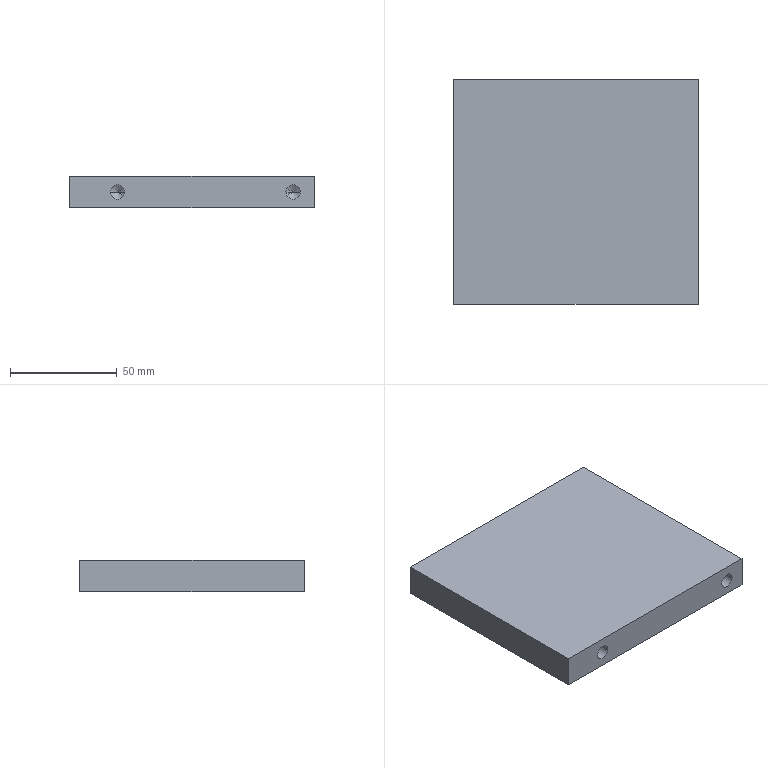Component | SolidWorks | FlipMechanismB-20-1 | 1 solid | 32 faces | box 115 x 105.4 x 15 mm | volume 177086 mm3 | cylinder 14 | cone 10 | plane 8 | commonest cylinder face diameters 6.8 x10 6 x4
build123d program:
from build123d import *

# Parameters (mm, degrees)
SKETCH1_W             = 115
SKETCH1_H             = 105.4
EXTRUDE1_DEPTH        = 7.5
M8_TAPPED_HOLE1_D     = 6.8
M8_TAPPED_HOLE1_DEPTH = 22.25
M8_TAPPED_HOLE1_TIP   = 2.043
SKETCH3_R             = 3
CUT_EXTRUDE1_DEPTH    = 10
M8_TAPPED_HOLE2_D     = 6.8
M8_TAPPED_HOLE2_DEPTH = 22.25
M8_TAPPED_HOLE2_TIP   = 2.043


with BuildPart() as part:
    # Sketch1 → Extrude1 (new, symmetric)
    with BuildSketch(Plane(origin=(0, 0, 0), x_dir=(1, 0, 0), z_dir=(0, 1, 0))):
        Rectangle(SKETCH1_W, SKETCH1_H)
    extrude(amount=EXTRUDE1_DEPTH, both=True)

    # M8 Tapped Hole1
    with Locations(Plane(origin=(0, 0, -52.7), x_dir=(-1, 0, 0), z_dir=(0, 0, -1))):
        with Locations((-47.5, 0), (47.5, 0), (0, 0)):
            Hole(M8_TAPPED_HOLE1_D / 2, depth=M8_TAPPED_HOLE1_DEPTH)
            with Locations((0, 0, -(M8_TAPPED_HOLE1_DEPTH + M8_TAPPED_HOLE1_TIP / 2))):  # 118° drill point
                Cone(0, M8_TAPPED_HOLE1_D / 2, M8_TAPPED_HOLE1_TIP, mode=Mode.SUBTRACT)

    # Sketch3 → Cut-Extrude1 (cut)
    with BuildSketch(Plane(origin=(0, 0, -52.7), x_dir=(-1, 0, 0), z_dir=(0, 0, -1))):
        with Locations((-27.5, 0)):
            Circle(SKETCH3_R)
        with Locations((27.5, 0)):
            Circle(SKETCH3_R)
    extrude(amount=-CUT_EXTRUDE1_DEPTH, mode=Mode.SUBTRACT)

    # M8 Tapped Hole2
    with Locations(Plane.XY.offset(52.7)):
        with Locations((-47.5, 0), (35, 0)):
            Hole(M8_TAPPED_HOLE2_D / 2, depth=M8_TAPPED_HOLE2_DEPTH)
            with Locations((0, 0, -(M8_TAPPED_HOLE2_DEPTH + M8_TAPPED_HOLE2_TIP / 2))):  # 118° drill point
                Cone(0, M8_TAPPED_HOLE2_D / 2, M8_TAPPED_HOLE2_TIP, mode=Mode.SUBTRACT)


solid = part.part

# Placed as in the assembly
solid = solid.moved(Location((12.5, 13.1, -289.5), (90, 0, -180)))
STEP:
#1=CARTESIAN_POINT('',(2.496,-0.6831,-11.398));
#2=VERTEX_POINT('',#1);
#3=CARTESIAN_POINT('',(2.228,-0.6831,-11.398));
#4=VERTEX_POINT('',#3);
#5=CARTESIAN_POINT('',(2.362,-0.6831,-11.398));
#6=DIRECTION('',(-0.,-1.,0.));
#7=DIRECTION('',(-1.,0.,0.));
#8=AXIS2_PLACEMENT_3D('',#5,#6,#7);
#9=CIRCLE('',#8,0.1339);
#10=EDGE_CURVE('',#2,#4,#9,.T.);
#11=ORIENTED_EDGE('',*,*,#10,.F.);
#12=CARTESIAN_POINT('',(2.496,-1.559,-11.398));
#13=VERTEX_POINT('',#12);
#14=CARTESIAN_POINT('',(2.496,-1.559,-11.398));
#15=DIRECTION('',(-0.,-1.,0.));
#16=VECTOR('',#15,39.37);
#17=LINE('',#14,#16);
#18=EDGE_CURVE('',#2,#13,#17,.T.);
#19=ORIENTED_EDGE('',*,*,#18,.T.);
#20=CARTESIAN_POINT('',(2.228,-1.559,-11.398));
#21=VERTEX_POINT('',#20);
#22=CARTESIAN_POINT('',(2.362,-1.559,-11.398));
#23=DIRECTION('',(-0.,-1.,0.));
#24=DIRECTION('',(-1.,0.,0.));
#25=AXIS2_PLACEMENT_3D('',#22,#23,#24);
#26=CIRCLE('',#25,0.1339);
#27=EDGE_CURVE('',#13,#21,#26,.T.);
#28=ORIENTED_EDGE('',*,*,#27,.T.);
#29=CARTESIAN_POINT('',(2.228,-1.559,-11.398));
#30=DIRECTION('',(-0.,-1.,0.));
#31=VECTOR('',#30,39.37);
#32=LINE('',#29,#31);
#33=EDGE_CURVE('',#4,#21,#32,.T.);
#34=ORIENTED_EDGE('',*,*,#33,.F.);
#35=EDGE_LOOP('',(#11,#19,#28,#34));
#36=FACE_OUTER_BOUND('',#35,.T.);
#37=CARTESIAN_POINT('',(2.362,-1.559,-11.398));
#38=DIRECTION('',(-0.,-1.,0.));
#39=DIRECTION('',(-1.,0.,0.));
#40=AXIS2_PLACEMENT_3D('',#37,#38,#39);
#41=CYLINDRICAL_SURFACE('',#40,0.1339);
#42=ADVANCED_FACE('',(#36),#41,.F.);
#43=CARTESIAN_POINT('',(2.362,-0.6026,-11.398));
#44=VERTEX_POINT('',#43);
#45=CARTESIAN_POINT('',(2.228,-0.6831,-11.398));
#46=DIRECTION('',(-0.8572,-0.515,0.));
#47=VECTOR('',#46,39.37);
#48=LINE('',#45,#47);
#49=EDGE_CURVE('',#44,#4,#48,.T.);
#50=ORIENTED_EDGE('',*,*,#49,.F.);
#51=CARTESIAN_POINT('',(2.496,-0.6831,-11.398));
#52=DIRECTION('',(0.8572,-0.515,-0.));
#53=VECTOR('',#52,39.37);
#54=LINE('',#51,#53);
#55=EDGE_CURVE('',#44,#2,#54,.T.);
#56=ORIENTED_EDGE('',*,*,#55,.T.);
#57=ORIENTED_EDGE('',*,*,#10,.T.);
#58=EDGE_LOOP('',(#50,#56,#57));
#59=FACE_OUTER_BOUND('',#58,.T.);
#60=CARTESIAN_POINT('',(2.362,-0.6831,-11.398));
#61=DIRECTION('',(-0.,-1.,0.));
#62=DIRECTION('',(-1.,0.,0.));
#63=AXIS2_PLACEMENT_3D('',#60,#61,#62);
#64=CONICAL_SURFACE('',#63,0.1339,1.03);
#65=ADVANCED_FACE('',(#59),#64,.F.);
#66=CARTESIAN_POINT('',(-0.752,-0.6831,-11.398));
#67=VERTEX_POINT('',#66);
#68=CARTESIAN_POINT('',(-1.02,-0.6831,-11.398));
#69=VERTEX_POINT('',#68);
#70=CARTESIAN_POINT('',(-0.8858,-0.6831,-11.398));
#71=DIRECTION('',(-0.,-1.,0.));
#72=DIRECTION('',(-1.,0.,0.));
#73=AXIS2_PLACEMENT_3D('',#70,#71,#72);
#74=CIRCLE('',#73,0.1339);
#75=EDGE_CURVE('',#67,#69,#74,.T.);
#76=ORIENTED_EDGE('',*,*,#75,.F.);
#77=CARTESIAN_POINT('',(-0.752,-1.559,-11.398));
#78=VERTEX_POINT('',#77);
#79=CARTESIAN_POINT('',(-0.752,-1.559,-11.398));
#80=DIRECTION('',(-0.,-1.,0.));
#81=VECTOR('',#80,39.37);
#82=LINE('',#79,#81);
#83=EDGE_CURVE('',#67,#78,#82,.T.);
#84=ORIENTED_EDGE('',*,*,#83,.T.);
#85=CARTESIAN_POINT('',(-1.02,-1.559,-11.398));
#86=VERTEX_POINT('',#85);
#87=CARTESIAN_POINT('',(-0.8858,-1.559,-11.398));
#88=DIRECTION('',(-0.,-1.,0.));
#89=DIRECTION('',(-1.,0.,0.));
#90=AXIS2_PLACEMENT_3D('',#87,#88,#89);
#91=CIRCLE('',#90,0.1339);
#92=EDGE_CURVE('',#78,#86,#91,.T.);
#93=ORIENTED_EDGE('',*,*,#92,.T.);
#94=CARTESIAN_POINT('',(-1.02,-1.559,-11.398));
#95=DIRECTION('',(-0.,-1.,0.));
#96=VECTOR('',#95,39.37);
#97=LINE('',#94,#96);
#98=EDGE_CURVE('',#69,#86,#97,.T.);
#99=ORIENTED_EDGE('',*,*,#98,.F.);
#100=EDGE_LOOP('',(#76,#84,#93,#99));
#101=FACE_OUTER_BOUND('',#100,.T.);
#102=CARTESIAN_POINT('',(-0.8858,-1.559,-11.398));
#103=DIRECTION('',(-0.,-1.,0.));
#104=DIRECTION('',(-1.,0.,0.));
#105=AXIS2_PLACEMENT_3D('',#102,#103,#104);
#106=CYLINDRICAL_SURFACE('',#105,0.1339);
#107=ADVANCED_FACE('',(#101),#106,.F.);
#108=CARTESIAN_POINT('',(-0.8858,-0.6026,-11.398));
#109=VERTEX_POINT('',#108);
#110=CARTESIAN_POINT('',(-1.02,-0.6831,-11.398));
#111=DIRECTION('',(-0.8572,-0.515,0.));
#112=VECTOR('',#111,39.37);
#113=LINE('',#110,#112);
#114=EDGE_CURVE('',#109,#69,#113,.T.);
#115=ORIENTED_EDGE('',*,*,#114,.F.);
#116=CARTESIAN_POINT('',(-0.752,-0.6831,-11.398));
#117=DIRECTION('',(0.8572,-0.515,-0.));
#118=VECTOR('',#117,39.37);
#119=LINE('',#116,#118);
#120=EDGE_CURVE('',#109,#67,#119,.T.);
#121=ORIENTED_EDGE('',*,*,#120,.T.);
#122=ORIENTED_EDGE('',*,*,#75,.T.);
#123=EDGE_LOOP('',(#115,#121,#122));
#124=FACE_OUTER_BOUND('',#123,.T.);
#125=CARTESIAN_POINT('',(-0.8858,-0.6831,-11.398));
#126=DIRECTION('',(-0.,-1.,0.));
#127=DIRECTION('',(-1.,0.,0.));
#128=AXIS2_PLACEMENT_3D('',#125,#126,#127);
#129=CONICAL_SURFACE('',#128,0.1339,1.03);
#130=ADVANCED_FACE('',(#124),#129,.F.);
#131=CARTESIAN_POINT('',(1.457,2.197,-11.398));
#132=VERTEX_POINT('',#131);
#133=CARTESIAN_POINT('',(1.693,2.197,-11.398));
#134=VERTEX_POINT('',#133);
#135=CARTESIAN_POINT('',(1.575,2.197,-11.398));
#136=DIRECTION('',(0.,1.,-0.));
#137=DIRECTION('',(1.,0.,0.));
#138=AXIS2_PLACEMENT_3D('',#135,#136,#137);
#139=CIRCLE('',#138,0.1181);
#140=EDGE_CURVE('',#132,#134,#139,.T.);
#141=ORIENTED_EDGE('',*,*,#140,.F.);
#142=CARTESIAN_POINT('',(1.457,2.591,-11.398));
#143=VERTEX_POINT('',#142);
#144=CARTESIAN_POINT('',(1.457,2.197,-11.398));
#145=DIRECTION('',(0.,1.,-0.));
#146=VECTOR('',#145,39.37);
#147=LINE('',#144,#146);
#148=EDGE_CURVE('',#132,#143,#147,.T.);
#149=ORIENTED_EDGE('',*,*,#148,.T.);
#150=CARTESIAN_POINT('',(1.693,2.591,-11.398));
#151=VERTEX_POINT('',#150);
#152=CARTESIAN_POINT('',(1.575,2.591,-11.398));
#153=DIRECTION('',(0.,1.,-0.));
#154=DIRECTION('',(1.,0.,0.));
#155=AXIS2_PLACEMENT_3D('',#152,#153,#154);
#156=CIRCLE('',#155,0.1181);
#157=EDGE_CURVE('',#143,#151,#156,.T.);
#158=ORIENTED_EDGE('',*,*,#157,.T.);
#159=CARTESIAN_POINT('',(1.693,2.197,-11.398));
#160=DIRECTION('',(0.,1.,-0.));
#161=VECTOR('',#160,39.37);
#162=LINE('',#159,#161);
#163=EDGE_CURVE('',#134,#151,#162,.T.);
#164=ORIENTED_EDGE('',*,*,#163,.F.);
#165=EDGE_LOOP('',(#141,#149,#158,#164));
#166=FACE_OUTER_BOUND('',#165,.T.);
#167=CARTESIAN_POINT('',(1.575,2.197,-11.398));
#168=DIRECTION('',(0.,1.,-0.));
#169=DIRECTION('',(1.,0.,0.));
#170=AXIS2_PLACEMENT_3D('',#167,#168,#169);
#171=CYLINDRICAL_SURFACE('',#170,0.1181);
#172=ADVANCED_FACE('',(#166),#171,.F.);
#173=CARTESIAN_POINT('',(-0.7087,2.197,-11.398));
#174=VERTEX_POINT('',#173);
#175=CARTESIAN_POINT('',(-0.4724,2.197,-11.398));
#176=VERTEX_POINT('',#175);
#177=CARTESIAN_POINT('',(-0.5906,2.197,-11.398));
#178=DIRECTION('',(0.,1.,-0.));
#179=DIRECTION('',(1.,0.,0.));
#180=AXIS2_PLACEMENT_3D('',#177,#178,#179);
#181=CIRCLE('',#180,0.1181);
#182=EDGE_CURVE('',#174,#176,#181,.T.);
#183=ORIENTED_EDGE('',*,*,#182,.F.);
#184=CARTESIAN_POINT('',(-0.7087,2.591,-11.398));
#185=VERTEX_POINT('',#184);
#186=CARTESIAN_POINT('',(-0.7087,2.197,-11.398));
#187=DIRECTION('',(0.,1.,-0.));
#188=VECTOR('',#187,39.37);
#189=LINE('',#186,#188);
#190=EDGE_CURVE('',#174,#185,#189,.T.);
#191=ORIENTED_EDGE('',*,*,#190,.T.);
#192=CARTESIAN_POINT('',(-0.4724,2.591,-11.398));
#193=VERTEX_POINT('',#192);
#194=CARTESIAN_POINT('',(-0.5906,2.591,-11.398));
#195=DIRECTION('',(0.,1.,-0.));
#196=DIRECTION('',(1.,0.,0.));
#197=AXIS2_PLACEMENT_3D('',#194,#195,#196);
#198=CIRCLE('',#197,0.1181);
#199=EDGE_CURVE('',#185,#193,#198,.T.);
#200=ORIENTED_EDGE('',*,*,#199,.T.);
#201=CARTESIAN_POINT('',(-0.4724,2.197,-11.398));
#202=DIRECTION('',(0.,1.,-0.));
#203=VECTOR('',#202,39.37);
#204=LINE('',#201,#203);
#205=EDGE_CURVE('',#176,#193,#204,.T.);
#206=ORIENTED_EDGE('',*,*,#205,.F.);
#207=EDGE_LOOP('',(#183,#191,#200,#206));
#208=FACE_OUTER_BOUND('',#207,.T.);
#209=CARTESIAN_POINT('',(-0.5906,2.197,-11.398));
#210=DIRECTION('',(0.,1.,-0.));
#211=DIRECTION('',(1.,0.,0.));
#212=AXIS2_PLACEMENT_3D('',#209,#210,#211);
#213=CYLINDRICAL_SURFACE('',#212,0.1181);
#214=ADVANCED_FACE('',(#208),#213,.F.);
#215=CARTESIAN_POINT('',(-1.512,1.715,-11.398));
#216=VERTEX_POINT('',#215);
#217=CARTESIAN_POINT('',(-1.244,1.715,-11.398));
#218=VERTEX_POINT('',#217);
#219=CARTESIAN_POINT('',(-1.378,1.715,-11.398));
#220=DIRECTION('',(0.,1.,-0.));
#221=DIRECTION('',(1.,0.,0.));
#222=AXIS2_PLACEMENT_3D('',#219,#220,#221);
#223=CIRCLE('',#222,0.1339);
#224=EDGE_CURVE('',#216,#218,#223,.T.);
#225=ORIENTED_EDGE('',*,*,#224,.F.);
#226=CARTESIAN_POINT('',(-1.512,2.591,-11.398));
#227=VERTEX_POINT('',#226);
#228=CARTESIAN_POINT('',(-1.512,2.591,-11.398));
#229=DIRECTION('',(0.,1.,-0.));
#230=VECTOR('',#229,39.37);
#231=LINE('',#228,#230);
#232=EDGE_CURVE('',#216,#227,#231,.T.);
#233=ORIENTED_EDGE('',*,*,#232,.T.);
#234=CARTESIAN_POINT('',(-1.244,2.591,-11.398));
#235=VERTEX_POINT('',#234);
#236=CARTESIAN_POINT('',(-1.378,2.591,-11.398));
#237=DIRECTION('',(0.,1.,-0.));
#238=DIRECTION('',(1.,0.,0.));
#239=AXIS2_PLACEMENT_3D('',#236,#237,#238);
#240=CIRCLE('',#239,0.1339);
#241=EDGE_CURVE('',#227,#235,#240,.T.);
#242=ORIENTED_EDGE('',*,*,#241,.T.);
#243=CARTESIAN_POINT('',(-1.244,2.591,-11.398));
#244=DIRECTION('',(0.,1.,-0.));
#245=VECTOR('',#244,39.37);
#246=LINE('',#243,#245);
#247=EDGE_CURVE('',#218,#235,#246,.T.);
#248=ORIENTED_EDGE('',*,*,#247,.F.);
#249=EDGE_LOOP('',(#225,#233,#242,#248));
#250=FACE_OUTER_BOUND('',#249,.T.);
#251=CARTESIAN_POINT('',(-1.378,2.591,-11.398));
#252=DIRECTION('',(0.,1.,-0.));
#253=DIRECTION('',(1.,0.,0.));
#254=AXIS2_PLACEMENT_3D('',#251,#252,#253);
#255=CYLINDRICAL_SURFACE('',#254,0.1339);
#256=ADVANCED_FACE('',(#250),#255,.F.);
#257=CARTESIAN_POINT('',(-1.378,1.634,-11.398));
#258=VERTEX_POINT('',#257);
#259=CARTESIAN_POINT('',(-1.244,1.715,-11.398));
#260=DIRECTION('',(0.8572,0.515,-0.));
#261=VECTOR('',#260,39.37);
#262=LINE('',#259,#261);
#263=EDGE_CURVE('',#258,#218,#262,.T.);
#264=ORIENTED_EDGE('',*,*,#263,.F.);
#265=CARTESIAN_POINT('',(-1.512,1.715,-11.398));
#266=DIRECTION('',(-0.8572,0.515,-0.));
#267=VECTOR('',#266,39.37);
#268=LINE('',#265,#267);
#269=EDGE_CURVE('',#258,#216,#268,.T.);
#270=ORIENTED_EDGE('',*,*,#269,.T.);
#271=ORIENTED_EDGE('',*,*,#224,.T.);
#272=EDGE_LOOP('',(#264,#270,#271));
#273=FACE_OUTER_BOUND('',#272,.T.);
#274=CARTESIAN_POINT('',(-1.378,1.715,-11.398));
#275=DIRECTION('',(0.,1.,-0.));
#276=DIRECTION('',(1.,0.,0.));
#277=AXIS2_PLACEMENT_3D('',#274,#275,#276);
#278=CONICAL_SURFACE('',#277,0.1339,1.03);
#279=ADVANCED_FACE('',(#273),#278,.F.);
#280=CARTESIAN_POINT('',(2.228,1.715,-11.398));
#281=VERTEX_POINT('',#280);
#282=CARTESIAN_POINT('',(2.496,1.715,-11.398));
#283=VERTEX_POINT('',#282);
#284=CARTESIAN_POINT('',(2.362,1.715,-11.398));
#285=DIRECTION('',(0.,1.,-0.));
#286=DIRECTION('',(1.,0.,0.));
#287=AXIS2_PLACEMENT_3D('',#284,#285,#286);
#288=CIRCLE('',#287,0.1339);
#289=EDGE_CURVE('',#281,#283,#288,.T.);
#290=ORIENTED_EDGE('',*,*,#289,.F.);
#291=CARTESIAN_POINT('',(2.228,2.591,-11.398));
#292=VERTEX_POINT('',#291);
#293=CARTESIAN_POINT('',(2.228,2.591,-11.398));
#294=DIRECTION('',(0.,1.,-0.));
#295=VECTOR('',#294,39.37);
#296=LINE('',#293,#295);
#297=EDGE_CURVE('',#281,#292,#296,.T.);
#298=ORIENTED_EDGE('',*,*,#297,.T.);
#299=CARTESIAN_POINT('',(2.496,2.591,-11.398));
#300=VERTEX_POINT('',#299);
#301=CARTESIAN_POINT('',(2.362,2.591,-11.398));
#302=DIRECTION('',(0.,1.,-0.));
#303=DIRECTION('',(1.,0.,0.));
#304=AXIS2_PLACEMENT_3D('',#301,#302,#303);
#305=CIRCLE('',#304,0.1339);
#306=EDGE_CURVE('',#292,#300,#305,.T.);
#307=ORIENTED_EDGE('',*,*,#306,.T.);
#308=CARTESIAN_POINT('',(2.496,2.591,-11.398));
#309=DIRECTION('',(0.,1.,-0.));
#310=VECTOR('',#309,39.37);
#311=LINE('',#308,#310);
#312=EDGE_CURVE('',#283,#300,#311,.T.);
#313=ORIENTED_EDGE('',*,*,#312,.F.);
#314=EDGE_LOOP('',(#290,#298,#307,#313));
#315=FACE_OUTER_BOUND('',#314,.T.);
#316=CARTESIAN_POINT('',(2.362,2.591,-11.398));
#317=DIRECTION('',(0.,1.,-0.));
#318=DIRECTION('',(1.,0.,0.));
#319=AXIS2_PLACEMENT_3D('',#316,#317,#318);
#320=CYLINDRICAL_SURFACE('',#319,0.1339);
#321=ADVANCED_FACE('',(#315),#320,.F.);
#322=CARTESIAN_POINT('',(2.362,1.634,-11.398));
#323=VERTEX_POINT('',#322);
#324=CARTESIAN_POINT('',(2.496,1.715,-11.398));
#325=DIRECTION('',(0.8572,0.515,-0.));
#326=VECTOR('',#325,39.37);
#327=LINE('',#324,#326);
#328=EDGE_CURVE('',#323,#283,#327,.T.);
#329=ORIENTED_EDGE('',*,*,#328,.F.);
#330=CARTESIAN_POINT('',(2.228,1.715,-11.398));
#331=DIRECTION('',(-0.8572,0.515,-0.));
#332=VECTOR('',#331,39.37);
#333=LINE('',#330,#332);
#334=EDGE_CURVE('',#323,#281,#333,.T.);
#335=ORIENTED_EDGE('',*,*,#334,.T.);
#336=ORIENTED_EDGE('',*,*,#289,.T.);
#337=EDGE_LOOP('',(#329,#335,#336));
#338=FACE_OUTER_BOUND('',#337,.T.);
#339=CARTESIAN_POINT('',(2.362,1.715,-11.398));
#340=DIRECTION('',(0.,1.,-0.));
#341=DIRECTION('',(1.,0.,0.));
#342=AXIS2_PLACEMENT_3D('',#339,#340,#341);
#343=CONICAL_SURFACE('',#342,0.1339,1.03);
#344=ADVANCED_FACE('',(#338),#343,.F.);
#345=CARTESIAN_POINT('',(0.3583,1.715,-11.398));
#346=VERTEX_POINT('',#345);
#347=CARTESIAN_POINT('',(0.626,1.715,-11.398));
#348=VERTEX_POINT('',#347);
#349=CARTESIAN_POINT('',(0.4921,1.715,-11.398));
#350=DIRECTION('',(0.,1.,-0.));
#351=DIRECTION('',(1.,0.,0.));
#352=AXIS2_PLACEMENT_3D('',#349,#350,#351);
#353=CIRCLE('',#352,0.1339);
#354=EDGE_CURVE('',#346,#348,#353,.T.);
#355=ORIENTED_EDGE('',*,*,#354,.F.);
#356=CARTESIAN_POINT('',(0.3583,2.591,-11.398));
#357=VERTEX_POINT('',#356);
#358=CARTESIAN_POINT('',(0.3583,2.591,-11.398));
#359=DIRECTION('',(0.,1.,-0.));
#360=VECTOR('',#359,39.37);
#361=LINE('',#358,#360);
#362=EDGE_CURVE('',#346,#357,#361,.T.);
#363=ORIENTED_EDGE('',*,*,#362,.T.);
#364=CARTESIAN_POINT('',(0.626,2.591,-11.398));
#365=VERTEX_POINT('',#364);
#366=CARTESIAN_POINT('',(0.4921,2.591,-11.398));
#367=DIRECTION('',(0.,1.,-0.));
#368=DIRECTION('',(1.,0.,0.));
#369=AXIS2_PLACEMENT_3D('',#366,#367,#368);
#370=CIRCLE('',#369,0.1339);
#371=EDGE_CURVE('',#357,#365,#370,.T.);
#372=ORIENTED_EDGE('',*,*,#371,.T.);
#373=CARTESIAN_POINT('',(0.626,2.591,-11.398));
#374=DIRECTION('',(0.,1.,-0.));
#375=VECTOR('',#374,39.37);
#376=LINE('',#373,#375);
#377=EDGE_CURVE('',#348,#365,#376,.T.);
#378=ORIENTED_EDGE('',*,*,#377,.F.);
#379=EDGE_LOOP('',(#355,#363,#372,#378));
#380=FACE_OUTER_BOUND('',#379,.T.);
#381=CARTESIAN_POINT('',(0.4921,2.591,-11.398));
#382=DIRECTION('',(0.,1.,-0.));
#383=DIRECTION('',(1.,0.,0.));
#384=AXIS2_PLACEMENT_3D('',#381,#382,#383);
#385=CYLINDRICAL_SURFACE('',#384,0.1339);
#386=ADVANCED_FACE('',(#380),#385,.F.);
#387=CARTESIAN_POINT('',(0.4921,1.634,-11.398));
#388=VERTEX_POINT('',#387);
#389=CARTESIAN_POINT('',(0.626,1.715,-11.398));
#390=DIRECTION('',(0.8572,0.515,-0.));
#391=VECTOR('',#390,39.37);
#392=LINE('',#389,#391);
#393=EDGE_CURVE('',#388,#348,#392,.T.);
#394=ORIENTED_EDGE('',*,*,#393,.F.);
#395=CARTESIAN_POINT('',(0.3583,1.715,-11.398));
#396=DIRECTION('',(-0.8572,0.515,-0.));
#397=VECTOR('',#396,39.37);
#398=LINE('',#395,#397);
#399=EDGE_CURVE('',#388,#346,#398,.T.);
#400=ORIENTED_EDGE('',*,*,#399,.T.);
#401=ORIENTED_EDGE('',*,*,#354,.T.);
#402=EDGE_LOOP('',(#394,#400,#401));
#403=FACE_OUTER_BOUND('',#402,.T.);
#404=CARTESIAN_POINT('',(0.4921,1.715,-11.398));
#405=DIRECTION('',(0.,1.,-0.));
#406=DIRECTION('',(1.,0.,0.));
#407=AXIS2_PLACEMENT_3D('',#404,#405,#406);
#408=CONICAL_SURFACE('',#407,0.1339,1.03);
#409=ADVANCED_FACE('',(#403),#408,.F.);
#410=CARTESIAN_POINT('',(2.756,2.591,-11.102));
#411=VERTEX_POINT('',#410);
#412=CARTESIAN_POINT('',(2.756,-1.559,-11.102));
#413=VERTEX_POINT('',#412);
#414=CARTESIAN_POINT('',(2.756,2.591,-11.102));
#415=DIRECTION('',(-0.,-1.,0.));
#416=VECTOR('',#415,39.37);
#417=LINE('',#414,#416);
#418=EDGE_CURVE('',#411,#413,#417,.T.);
#419=ORIENTED_EDGE('',*,*,#418,.T.);
#420=CARTESIAN_POINT('',(2.756,-1.559,-11.693));
#421=VERTEX_POINT('',#420);
#422=CARTESIAN_POINT('',(2.756,-1.559,-11.693));
#423=DIRECTION('',(0.,0.,1.));
#424=VECTOR('',#423,39.37);
#425=LINE('',#422,#424);
#426=EDGE_CURVE('',#421,#413,#425,.T.);
#427=ORIENTED_EDGE('',*,*,#426,.F.);
#428=CARTESIAN_POINT('',(2.756,2.591,-11.693));
#429=VERTEX_POINT('',#428);
#430=CARTESIAN_POINT('',(2.756,2.591,-11.693));
#431=DIRECTION('',(-0.,-1.,0.));
#432=VECTOR('',#431,39.37);
#433=LINE('',#430,#432);
#434=EDGE_CURVE('',#429,#421,#433,.T.);
#435=ORIENTED_EDGE('',*,*,#434,.F.);
#436=CARTESIAN_POINT('',(2.756,2.591,-11.693));
#437=DIRECTION('',(0.,0.,1.));
#438=VECTOR('',#437,39.37);
#439=LINE('',#436,#438);
#440=EDGE_CURVE('',#429,#411,#439,.T.);
#441=ORIENTED_EDGE('',*,*,#440,.T.);
#442=EDGE_LOOP('',(#419,#427,#435,#441));
#443=FACE_OUTER_BOUND('',#442,.T.);
#444=CARTESIAN_POINT('',(2.756,2.591,-11.693));
#445=DIRECTION('',(-1.,0.,0.));
#446=DIRECTION('',(0.,1.,-0.));
#447=AXIS2_PLACEMENT_3D('',#444,#445,#446);
#448=PLANE('',#447);
#449=ADVANCED_FACE('',(#443),#448,.F.);
#450=CARTESIAN_POINT('',(2.362,-1.559,-11.398));
#451=DIRECTION('',(-0.,-1.,0.));
#452=DIRECTION('',(-1.,0.,0.));
#453=AXIS2_PLACEMENT_3D('',#450,#451,#452);
#454=CIRCLE('',#453,0.1339);
#455=EDGE_CURVE('',#21,#13,#454,.T.);
#456=ORIENTED_EDGE('',*,*,#455,.F.);
#457=ORIENTED_EDGE('',*,*,#27,.F.);
#458=EDGE_LOOP('',(#456,#457));
#459=FACE_BOUND('',#458,.T.);
#460=CARTESIAN_POINT('',(-0.8858,-1.559,-11.398));
#461=DIRECTION('',(-0.,-1.,0.));
#462=DIRECTION('',(-1.,0.,0.));
#463=AXIS2_PLACEMENT_3D('',#460,#461,#462);
#464=CIRCLE('',#463,0.1339);
#465=EDGE_CURVE('',#86,#78,#464,.T.);
#466=ORIENTED_EDGE('',*,*,#465,.F.);
#467=ORIENTED_EDGE('',*,*,#92,.F.);
#468=EDGE_LOOP('',(#466,#467));
#469=FACE_BOUND('',#468,.T.);
#470=CARTESIAN_POINT('',(-1.772,-1.559,-11.102));
#471=VERTEX_POINT('',#470);
#472=CARTESIAN_POINT('',(2.756,-1.559,-11.102));
#473=DIRECTION('',(-1.,0.,0.));
#474=VECTOR('',#473,39.37);
#475=LINE('',#472,#474);
#476=EDGE_CURVE('',#413,#471,#475,.T.);
#477=ORIENTED_EDGE('',*,*,#476,.T.);
#478=CARTESIAN_POINT('',(-1.772,-1.559,-11.693));
#479=VERTEX_POINT('',#478);
#480=CARTESIAN_POINT('',(-1.772,-1.559,-11.693));
#481=DIRECTION('',(0.,0.,1.));
#482=VECTOR('',#481,39.37);
#483=LINE('',#480,#482);
#484=EDGE_CURVE('',#479,#471,#483,.T.);
#485=ORIENTED_EDGE('',*,*,#484,.F.);
#486=CARTESIAN_POINT('',(2.756,-1.559,-11.693));
#487=DIRECTION('',(-1.,0.,0.));
#488=VECTOR('',#487,39.37);
#489=LINE('',#486,#488);
#490=EDGE_CURVE('',#421,#479,#489,.T.);
#491=ORIENTED_EDGE('',*,*,#490,.F.);
#492=ORIENTED_EDGE('',*,*,#426,.T.);
#493=EDGE_LOOP('',(#477,#485,#491,#492));
#494=FACE_OUTER_BOUND('',#493,.T.);
#495=CARTESIAN_POINT('',(2.756,-1.559,-11.693));
#496=DIRECTION('',(0.,1.,-0.));
#497=DIRECTION('',(1.,-0.,-0.));
#498=AXIS2_PLACEMENT_3D('',#495,#496,#497);
#499=PLANE('',#498);
#500=ADVANCED_FACE('',(#459,#469,#494),#499,.F.);
#501=CARTESIAN_POINT('',(-1.772,2.591,-11.102));
#502=VERTEX_POINT('',#501);
#503=CARTESIAN_POINT('',(-1.772,2.591,-11.102));
#504=DIRECTION('',(0.,1.,-0.));
#505=VECTOR('',#504,39.37);
#506=LINE('',#503,#505);
#507=EDGE_CURVE('',#471,#502,#506,.T.);
#508=ORIENTED_EDGE('',*,*,#507,.T.);
#509=CARTESIAN_POINT('',(-1.772,2.591,-11.693));
#510=VERTEX_POINT('',#509);
#511=CARTESIAN_POINT('',(-1.772,2.591,-11.693));
#512=DIRECTION('',(0.,0.,1.));
#513=VECTOR('',#512,39.37);
#514=LINE('',#511,#513);
#515=EDGE_CURVE('',#510,#502,#514,.T.);
#516=ORIENTED_EDGE('',*,*,#515,.F.);
#517=CARTESIAN_POINT('',(-1.772,2.591,-11.693));
#518=DIRECTION('',(0.,1.,-0.));
#519=VECTOR('',#518,39.37);
#520=LINE('',#517,#519);
#521=EDGE_CURVE('',#479,#510,#520,.T.);
#522=ORIENTED_EDGE('',*,*,#521,.F.);
#523=ORIENTED_EDGE('',*,*,#484,.T.);
#524=EDGE_LOOP('',(#508,#516,#522,#523));
#525=FACE_OUTER_BOUND('',#524,.T.);
#526=CARTESIAN_POINT('',(-1.772,2.591,-11.693));
#527=DIRECTION('',(1.,-0.,-0.));
#528=DIRECTION('',(-0.,-1.,0.));
#529=AXIS2_PLACEMENT_3D('',#526,#527,#528);
#530=PLANE('',#529);
#531=ADVANCED_FACE('',(#525),#530,.F.);
#532=CARTESIAN_POINT('',(1.575,2.591,-11.398));
#533=DIRECTION('',(0.,1.,-0.));
#534=DIRECTION('',(1.,0.,0.));
#535=AXIS2_PLACEMENT_3D('',#532,#533,#534);
#536=CIRCLE('',#535,0.1181);
#537=EDGE_CURVE('',#151,#143,#536,.T.);
#538=ORIENTED_EDGE('',*,*,#537,.F.);
#539=ORIENTED_EDGE('',*,*,#157,.F.);
#540=EDGE_LOOP('',(#538,#539));
#541=FACE_BOUND('',#540,.T.);
#542=CARTESIAN_POINT('',(-0.5906,2.591,-11.398));
#543=DIRECTION('',(0.,1.,-0.));
#544=DIRECTION('',(1.,0.,0.));
#545=AXIS2_PLACEMENT_3D('',#542,#543,#544);
#546=CIRCLE('',#545,0.1181);
#547=EDGE_CURVE('',#193,#185,#546,.T.);
#548=ORIENTED_EDGE('',*,*,#547,.F.);
#549=ORIENTED_EDGE('',*,*,#199,.F.);
#550=EDGE_LOOP('',(#548,#549));
#551=FACE_BOUND('',#550,.T.);
#552=CARTESIAN_POINT('',(-1.378,2.591,-11.398));
#553=DIRECTION('',(0.,1.,-0.));
#554=DIRECTION('',(1.,0.,0.));
#555=AXIS2_PLACEMENT_3D('',#552,#553,#554);
#556=CIRCLE('',#555,0.1339);
#557=EDGE_CURVE('',#235,#227,#556,.T.);
#558=ORIENTED_EDGE('',*,*,#557,.F.);
#559=ORIENTED_EDGE('',*,*,#241,.F.);
#560=EDGE_LOOP('',(#558,#559));
#561=FACE_BOUND('',#560,.T.);
#562=CARTESIAN_POINT('',(2.362,2.591,-11.398));
#563=DIRECTION('',(0.,1.,-0.));
#564=DIRECTION('',(1.,0.,0.));
#565=AXIS2_PLACEMENT_3D('',#562,#563,#564);
#566=CIRCLE('',#565,0.1339);
#567=EDGE_CURVE('',#300,#292,#566,.T.);
#568=ORIENTED_EDGE('',*,*,#567,.F.);
#569=ORIENTED_EDGE('',*,*,#306,.F.);
#570=EDGE_LOOP('',(#568,#569));
#571=FACE_BOUND('',#570,.T.);
#572=CARTESIAN_POINT('',(0.4921,2.591,-11.398));
#573=DIRECTION('',(0.,1.,-0.));
#574=DIRECTION('',(1.,0.,0.));
#575=AXIS2_PLACEMENT_3D('',#572,#573,#574);
#576=CIRCLE('',#575,0.1339);
#577=EDGE_CURVE('',#365,#357,#576,.T.);
#578=ORIENTED_EDGE('',*,*,#577,.F.);
#579=ORIENTED_EDGE('',*,*,#371,.F.);
#580=EDGE_LOOP('',(#578,#579));
#581=FACE_BOUND('',#580,.T.);
#582=CARTESIAN_POINT('',(2.756,2.591,-11.102));
#583=DIRECTION('',(1.,-0.,-0.));
#584=VECTOR('',#583,39.37);
#585=LINE('',#582,#584);
#586=EDGE_CURVE('',#502,#411,#585,.T.);
#587=ORIENTED_EDGE('',*,*,#586,.T.);
#588=ORIENTED_EDGE('',*,*,#440,.F.);
#589=CARTESIAN_POINT('',(2.756,2.591,-11.693));
#590=DIRECTION('',(1.,-0.,-0.));
#591=VECTOR('',#590,39.37);
#592=LINE('',#589,#591);
#593=EDGE_CURVE('',#510,#429,#592,.T.);
#594=ORIENTED_EDGE('',*,*,#593,.F.);
#595=ORIENTED_EDGE('',*,*,#515,.T.);
#596=EDGE_LOOP('',(#587,#588,#594,#595));
#597=FACE_OUTER_BOUND('',#596,.T.);
#598=CARTESIAN_POINT('',(2.756,2.591,-11.693));
#599=DIRECTION('',(-0.,-1.,0.));
#600=DIRECTION('',(-1.,0.,0.));
#601=AXIS2_PLACEMENT_3D('',#598,#599,#600);
#602=PLANE('',#601);
#603=ADVANCED_FACE('',(#541,#551,#561,#571,#581,#597),#602,.F.);
#604=ORIENTED_EDGE('',*,*,#434,.T.);
#605=ORIENTED_EDGE('',*,*,#490,.T.);
#606=ORIENTED_EDGE('',*,*,#521,.T.);
#607=ORIENTED_EDGE('',*,*,#593,.T.);
#608=EDGE_LOOP('',(#604,#605,#606,#607));
#609=FACE_OUTER_BOUND('',#608,.T.);
#610=CARTESIAN_POINT('',(0.4921,0.5157,-11.693));
#611=DIRECTION('',(-0.,-0.,-1.));
#612=DIRECTION('',(-0.,-1.,0.));
#613=AXIS2_PLACEMENT_3D('',#610,#611,#612);
#614=PLANE('',#613);
#615=ADVANCED_FACE('',(#609),#614,.T.);
#616=ORIENTED_EDGE('',*,*,#418,.F.);
#617=ORIENTED_EDGE('',*,*,#586,.F.);
#618=ORIENTED_EDGE('',*,*,#507,.F.);
#619=ORIENTED_EDGE('',*,*,#476,.F.);
#620=EDGE_LOOP('',(#616,#617,#618,#619));
#621=FACE_OUTER_BOUND('',#620,.T.);
#622=CARTESIAN_POINT('',(0.4921,0.5157,-11.102));
#623=DIRECTION('',(-0.,-0.,-1.));
#624=DIRECTION('',(-0.,-1.,0.));
#625=AXIS2_PLACEMENT_3D('',#622,#623,#624);
#626=PLANE('',#625);
#627=ADVANCED_FACE('',(#621),#626,.F.);
#628=ORIENTED_EDGE('',*,*,#399,.F.);
#629=ORIENTED_EDGE('',*,*,#393,.T.);
#630=CARTESIAN_POINT('',(0.4921,1.715,-11.398));
#631=DIRECTION('',(0.,1.,-0.));
#632=DIRECTION('',(1.,0.,0.));
#633=AXIS2_PLACEMENT_3D('',#630,#631,#632);
#634=CIRCLE('',#633,0.1339);
#635=EDGE_CURVE('',#348,#346,#634,.T.);
#636=ORIENTED_EDGE('',*,*,#635,.T.);
#637=EDGE_LOOP('',(#628,#629,#636));
#638=FACE_OUTER_BOUND('',#637,.T.);
#639=CARTESIAN_POINT('',(0.4921,1.715,-11.398));
#640=DIRECTION('',(0.,1.,-0.));
#641=DIRECTION('',(1.,0.,0.));
#642=AXIS2_PLACEMENT_3D('',#639,#640,#641);
#643=CONICAL_SURFACE('',#642,0.1339,1.03);
#644=ADVANCED_FACE('',(#638),#643,.F.);
#645=ORIENTED_EDGE('',*,*,#362,.F.);
#646=ORIENTED_EDGE('',*,*,#635,.F.);
#647=ORIENTED_EDGE('',*,*,#377,.T.);
#648=ORIENTED_EDGE('',*,*,#577,.T.);
#649=EDGE_LOOP('',(#645,#646,#647,#648));
#650=FACE_OUTER_BOUND('',#649,.T.);
#651=CARTESIAN_POINT('',(0.4921,2.591,-11.398));
#652=DIRECTION('',(0.,1.,-0.));
#653=DIRECTION('',(1.,0.,0.));
#654=AXIS2_PLACEMENT_3D('',#651,#652,#653);
#655=CYLINDRICAL_SURFACE('',#654,0.1339);
#656=ADVANCED_FACE('',(#650),#655,.F.);
#657=ORIENTED_EDGE('',*,*,#334,.F.);
#658=ORIENTED_EDGE('',*,*,#328,.T.);
#659=CARTESIAN_POINT('',(2.362,1.715,-11.398));
#660=DIRECTION('',(0.,1.,-0.));
#661=DIRECTION('',(1.,0.,0.));
#662=AXIS2_PLACEMENT_3D('',#659,#660,#661);
#663=CIRCLE('',#662,0.1339);
#664=EDGE_CURVE('',#283,#281,#663,.T.);
#665=ORIENTED_EDGE('',*,*,#664,.T.);
#666=EDGE_LOOP('',(#657,#658,#665));
#667=FACE_OUTER_BOUND('',#666,.T.);
#668=CARTESIAN_POINT('',(2.362,1.715,-11.398));
#669=DIRECTION('',(0.,1.,-0.));
#670=DIRECTION('',(1.,0.,0.));
#671=AXIS2_PLACEMENT_3D('',#668,#669,#670);
#672=CONICAL_SURFACE('',#671,0.1339,1.03);
#673=ADVANCED_FACE('',(#667),#672,.F.);
#674=ORIENTED_EDGE('',*,*,#297,.F.);
#675=ORIENTED_EDGE('',*,*,#664,.F.);
#676=ORIENTED_EDGE('',*,*,#312,.T.);
#677=ORIENTED_EDGE('',*,*,#567,.T.);
#678=EDGE_LOOP('',(#674,#675,#676,#677));
#679=FACE_OUTER_BOUND('',#678,.T.);
#680=CARTESIAN_POINT('',(2.362,2.591,-11.398));
#681=DIRECTION('',(0.,1.,-0.));
#682=DIRECTION('',(1.,0.,0.));
#683=AXIS2_PLACEMENT_3D('',#680,#681,#682);
#684=CYLINDRICAL_SURFACE('',#683,0.1339);
#685=ADVANCED_FACE('',(#679),#684,.F.);
#686=ORIENTED_EDGE('',*,*,#269,.F.);
#687=ORIENTED_EDGE('',*,*,#263,.T.);
#688=CARTESIAN_POINT('',(-1.378,1.715,-11.398));
#689=DIRECTION('',(0.,1.,-0.));
#690=DIRECTION('',(1.,0.,0.));
#691=AXIS2_PLACEMENT_3D('',#688,#689,#690);
#692=CIRCLE('',#691,0.1339);
#693=EDGE_CURVE('',#218,#216,#692,.T.);
#694=ORIENTED_EDGE('',*,*,#693,.T.);
#695=EDGE_LOOP('',(#686,#687,#694));
#696=FACE_OUTER_BOUND('',#695,.T.);
#697=CARTESIAN_POINT('',(-1.378,1.715,-11.398));
#698=DIRECTION('',(0.,1.,-0.));
#699=DIRECTION('',(1.,0.,0.));
#700=AXIS2_PLACEMENT_3D('',#697,#698,#699);
#701=CONICAL_SURFACE('',#700,0.1339,1.03);
#702=ADVANCED_FACE('',(#696),#701,.F.);
#703=ORIENTED_EDGE('',*,*,#232,.F.);
#704=ORIENTED_EDGE('',*,*,#693,.F.);
#705=ORIENTED_EDGE('',*,*,#247,.T.);
#706=ORIENTED_EDGE('',*,*,#557,.T.);
#707=EDGE_LOOP('',(#703,#704,#705,#706));
#708=FACE_OUTER_BOUND('',#707,.T.);
#709=CARTESIAN_POINT('',(-1.378,2.591,-11.398));
#710=DIRECTION('',(0.,1.,-0.));
#711=DIRECTION('',(1.,0.,0.));
#712=AXIS2_PLACEMENT_3D('',#709,#710,#711);
#713=CYLINDRICAL_SURFACE('',#712,0.1339);
#714=ADVANCED_FACE('',(#708),#713,.F.);
#715=ORIENTED_EDGE('',*,*,#190,.F.);
#716=CARTESIAN_POINT('',(-0.5906,2.197,-11.398));
#717=DIRECTION('',(0.,1.,-0.));
#718=DIRECTION('',(1.,0.,0.));
#719=AXIS2_PLACEMENT_3D('',#716,#717,#718);
#720=CIRCLE('',#719,0.1181);
#721=EDGE_CURVE('',#176,#174,#720,.T.);
#722=ORIENTED_EDGE('',*,*,#721,.F.);
#723=ORIENTED_EDGE('',*,*,#205,.T.);
#724=ORIENTED_EDGE('',*,*,#547,.T.);
#725=EDGE_LOOP('',(#715,#722,#723,#724));
#726=FACE_OUTER_BOUND('',#725,.T.);
#727=CARTESIAN_POINT('',(-0.5906,2.197,-11.398));
#728=DIRECTION('',(0.,1.,-0.));
#729=DIRECTION('',(1.,0.,0.));
#730=AXIS2_PLACEMENT_3D('',#727,#728,#729);
#731=CYLINDRICAL_SURFACE('',#730,0.1181);
#732=ADVANCED_FACE('',(#726),#731,.F.);
#733=ORIENTED_EDGE('',*,*,#721,.T.);
#734=ORIENTED_EDGE('',*,*,#182,.T.);
#735=EDGE_LOOP('',(#733,#734));
#736=FACE_OUTER_BOUND('',#735,.T.);
#737=CARTESIAN_POINT('',(-0.5906,2.197,-11.398));
#738=DIRECTION('',(0.,1.,-0.));
#739=DIRECTION('',(1.,-0.,-0.));
#740=AXIS2_PLACEMENT_3D('',#737,#738,#739);
#741=PLANE('',#740);
#742=ADVANCED_FACE('',(#736),#741,.T.);
#743=ORIENTED_EDGE('',*,*,#148,.F.);
#744=CARTESIAN_POINT('',(1.575,2.197,-11.398));
#745=DIRECTION('',(0.,1.,-0.));
#746=DIRECTION('',(1.,0.,0.));
#747=AXIS2_PLACEMENT_3D('',#744,#745,#746);
#748=CIRCLE('',#747,0.1181);
#749=EDGE_CURVE('',#134,#132,#748,.T.);
#750=ORIENTED_EDGE('',*,*,#749,.F.);
#751=ORIENTED_EDGE('',*,*,#163,.T.);
#752=ORIENTED_EDGE('',*,*,#537,.T.);
#753=EDGE_LOOP('',(#743,#750,#751,#752));
#754=FACE_OUTER_BOUND('',#753,.T.);
#755=CARTESIAN_POINT('',(1.575,2.197,-11.398));
#756=DIRECTION('',(0.,1.,-0.));
#757=DIRECTION('',(1.,0.,0.));
#758=AXIS2_PLACEMENT_3D('',#755,#756,#757);
#759=CYLINDRICAL_SURFACE('',#758,0.1181);
#760=ADVANCED_FACE('',(#754),#759,.F.);
#761=ORIENTED_EDGE('',*,*,#749,.T.);
#762=ORIENTED_EDGE('',*,*,#140,.T.);
#763=EDGE_LOOP('',(#761,#762));
#764=FACE_OUTER_BOUND('',#763,.T.);
#765=CARTESIAN_POINT('',(1.575,2.197,-11.398));
#766=DIRECTION('',(0.,1.,-0.));
#767=DIRECTION('',(1.,-0.,-0.));
#768=AXIS2_PLACEMENT_3D('',#765,#766,#767);
#769=PLANE('',#768);
#770=ADVANCED_FACE('',(#764),#769,.T.);
#771=ORIENTED_EDGE('',*,*,#120,.F.);
#772=ORIENTED_EDGE('',*,*,#114,.T.);
#773=CARTESIAN_POINT('',(-0.8858,-0.6831,-11.398));
#774=DIRECTION('',(-0.,-1.,0.));
#775=DIRECTION('',(-1.,0.,0.));
#776=AXIS2_PLACEMENT_3D('',#773,#774,#775);
#777=CIRCLE('',#776,0.1339);
#778=EDGE_CURVE('',#69,#67,#777,.T.);
#779=ORIENTED_EDGE('',*,*,#778,.T.);
#780=EDGE_LOOP('',(#771,#772,#779));
#781=FACE_OUTER_BOUND('',#780,.T.);
#782=CARTESIAN_POINT('',(-0.8858,-0.6831,-11.398));
#783=DIRECTION('',(-0.,-1.,0.));
#784=DIRECTION('',(-1.,0.,0.));
#785=AXIS2_PLACEMENT_3D('',#782,#783,#784);
#786=CONICAL_SURFACE('',#785,0.1339,1.03);
#787=ADVANCED_FACE('',(#781),#786,.F.);
#788=ORIENTED_EDGE('',*,*,#83,.F.);
#789=ORIENTED_EDGE('',*,*,#778,.F.);
#790=ORIENTED_EDGE('',*,*,#98,.T.);
#791=ORIENTED_EDGE('',*,*,#465,.T.);
#792=EDGE_LOOP('',(#788,#789,#790,#791));
#793=FACE_OUTER_BOUND('',#792,.T.);
#794=CARTESIAN_POINT('',(-0.8858,-1.559,-11.398));
#795=DIRECTION('',(-0.,-1.,0.));
#796=DIRECTION('',(-1.,0.,0.));
#797=AXIS2_PLACEMENT_3D('',#794,#795,#796);
#798=CYLINDRICAL_SURFACE('',#797,0.1339);
#799=ADVANCED_FACE('',(#793),#798,.F.);
#800=ORIENTED_EDGE('',*,*,#55,.F.);
#801=ORIENTED_EDGE('',*,*,#49,.T.);
#802=CARTESIAN_POINT('',(2.362,-0.6831,-11.398));
#803=DIRECTION('',(-0.,-1.,0.));
#804=DIRECTION('',(-1.,0.,0.));
#805=AXIS2_PLACEMENT_3D('',#802,#803,#804);
#806=CIRCLE('',#805,0.1339);
#807=EDGE_CURVE('',#4,#2,#806,.T.);
#808=ORIENTED_EDGE('',*,*,#807,.T.);
#809=EDGE_LOOP('',(#800,#801,#808));
#810=FACE_OUTER_BOUND('',#809,.T.);
#811=CARTESIAN_POINT('',(2.362,-0.6831,-11.398));
#812=DIRECTION('',(-0.,-1.,0.));
#813=DIRECTION('',(-1.,0.,0.));
#814=AXIS2_PLACEMENT_3D('',#811,#812,#813);
#815=CONICAL_SURFACE('',#814,0.1339,1.03);
#816=ADVANCED_FACE('',(#810),#815,.F.);
#817=ORIENTED_EDGE('',*,*,#18,.F.);
#818=ORIENTED_EDGE('',*,*,#807,.F.);
#819=ORIENTED_EDGE('',*,*,#33,.T.);
#820=ORIENTED_EDGE('',*,*,#455,.T.);
#821=EDGE_LOOP('',(#817,#818,#819,#820));
#822=FACE_OUTER_BOUND('',#821,.T.);
#823=CARTESIAN_POINT('',(2.362,-1.559,-11.398));
#824=DIRECTION('',(-0.,-1.,0.));
#825=DIRECTION('',(-1.,0.,0.));
#826=AXIS2_PLACEMENT_3D('',#823,#824,#825);
#827=CYLINDRICAL_SURFACE('',#826,0.1339);
#828=ADVANCED_FACE('',(#822),#827,.F.);
#829=CLOSED_SHELL('',(#42,#65,#107,#130,#172,#214,#256,#279,#321,#344,#386,#409,#449,#500,#531,#603,#615,#627,#644,#656,#673,#685,#702,#714,#732,#742,#760,#770,#787,#799,#816,#828));
#830=MANIFOLD_SOLID_BREP('',#829);
#831=CARTESIAN_POINT('',(0.,0.,0.));
#832=DIRECTION('',(0.,0.,1.));
#833=DIRECTION('',(1.,0.,0.));
#834=AXIS2_PLACEMENT_3D('',#831,#832,#833);
#835=(LENGTH_UNIT()NAMED_UNIT(*)SI_UNIT($,.METRE.));
#836=LENGTH_MEASURE_WITH_UNIT(LENGTH_MEASURE(0.0254),#835);
#837=DIMENSIONAL_EXPONENTS(1.,0.,0.,0.,0.,0.,0.);
#838=(CONVERSION_BASED_UNIT('',#836)LENGTH_UNIT()NAMED_UNIT(#837));
#839=UNCERTAINTY_MEASURE_WITH_UNIT(LENGTH_MEASURE(0.00001),#838,'','');
#840=(NAMED_UNIT(*)PLANE_ANGLE_UNIT()SI_UNIT($,.RADIAN.));
#841=(NAMED_UNIT(*)SI_UNIT($,.STERADIAN.)SOLID_ANGLE_UNIT());
#842=(GEOMETRIC_REPRESENTATION_CONTEXT(3)GLOBAL_UNCERTAINTY_ASSIGNED_CONTEXT((#839))GLOBAL_UNIT_ASSIGNED_CONTEXT((#838,#840,#841))REPRESENTATION_CONTEXT('',''));
#843=ADVANCED_BREP_SHAPE_REPRESENTATION('',(#830,#834),#842);
#844=COLOUR_RGB('',0.7922,0.8196,0.9333);
#845=FILL_AREA_STYLE_COLOUR('',#844);
#846=FILL_AREA_STYLE('',(#845));
#847=SURFACE_STYLE_FILL_AREA(#846);
#848=SURFACE_SIDE_STYLE('',(#847));
#849=SURFACE_STYLE_USAGE(.BOTH.,#848);
#850=PRESENTATION_STYLE_ASSIGNMENT((#849));
#851=STYLED_ITEM('',(#850),#830);
#852=PRESENTATION_LAYER_ASSIGNMENT('','',(#851));
#853=(LENGTH_UNIT()NAMED_UNIT(*)SI_UNIT($,.METRE.));
#854=LENGTH_MEASURE_WITH_UNIT(LENGTH_MEASURE(0.0254),#853);
#855=DIMENSIONAL_EXPONENTS(1.,0.,0.,0.,0.,0.,0.);
#856=(CONVERSION_BASED_UNIT('',#854)LENGTH_UNIT()NAMED_UNIT(#855));
#857=UNCERTAINTY_MEASURE_WITH_UNIT(LENGTH_MEASURE(0.00001),#856,'','');
#858=(NAMED_UNIT(*)PLANE_ANGLE_UNIT()SI_UNIT($,.RADIAN.));
#859=(NAMED_UNIT(*)SI_UNIT($,.STERADIAN.)SOLID_ANGLE_UNIT());
#860=(GEOMETRIC_REPRESENTATION_CONTEXT(3)GLOBAL_UNCERTAINTY_ASSIGNED_CONTEXT((#857))GLOBAL_UNIT_ASSIGNED_CONTEXT((#856,#858,#859))REPRESENTATION_CONTEXT('',''));
#861=MECHANICAL_DESIGN_GEOMETRIC_PRESENTATION_REPRESENTATION('',(#851),#860);